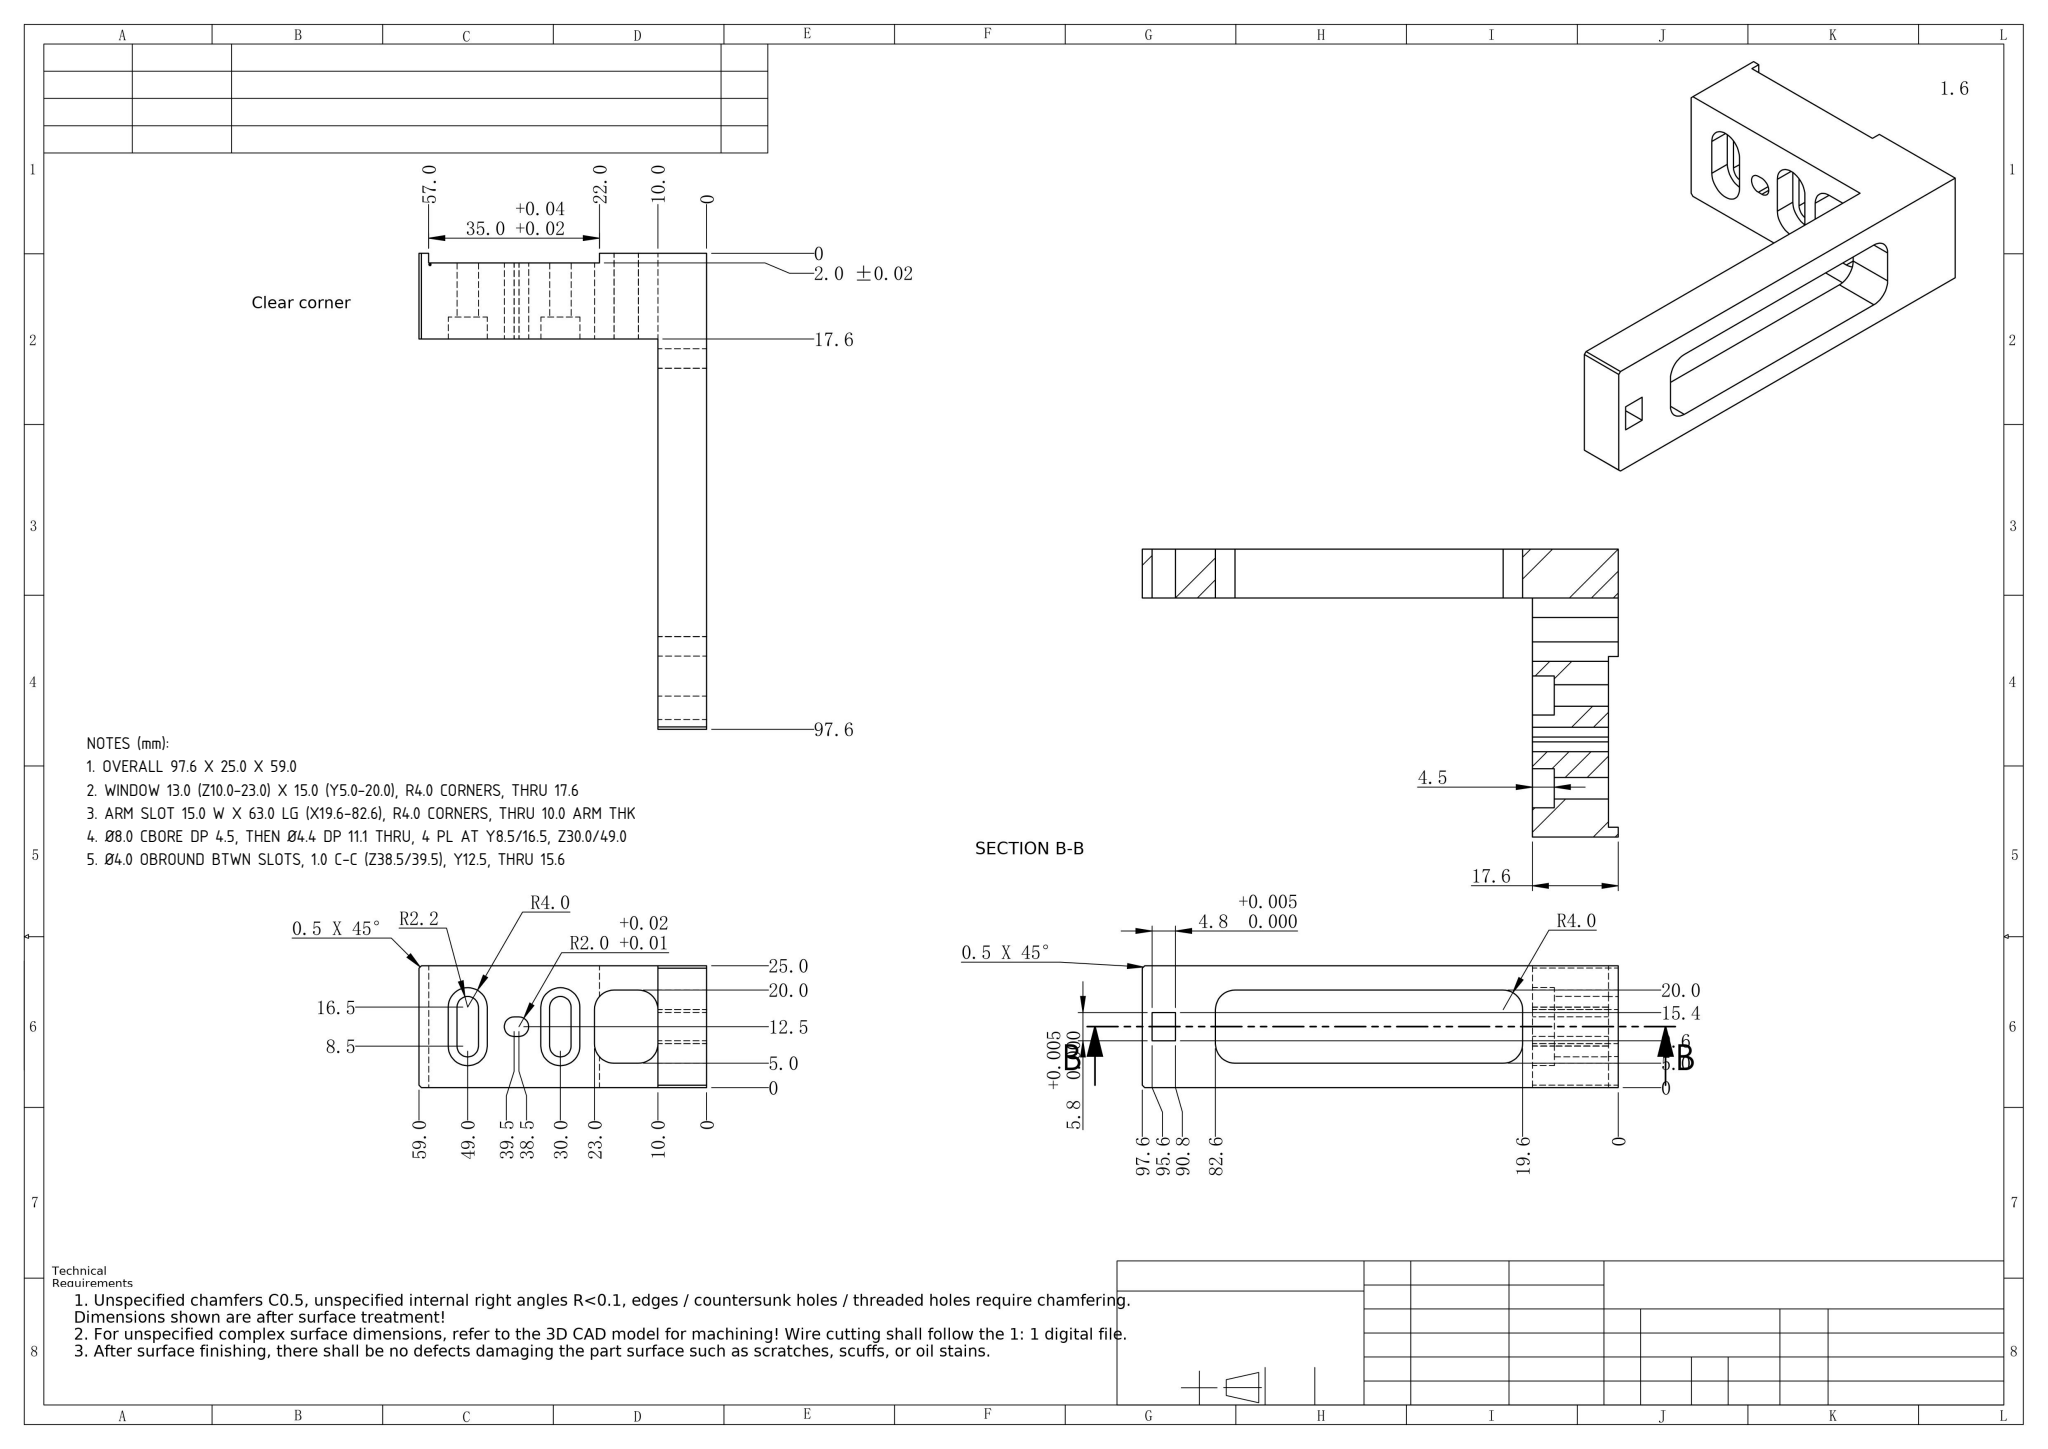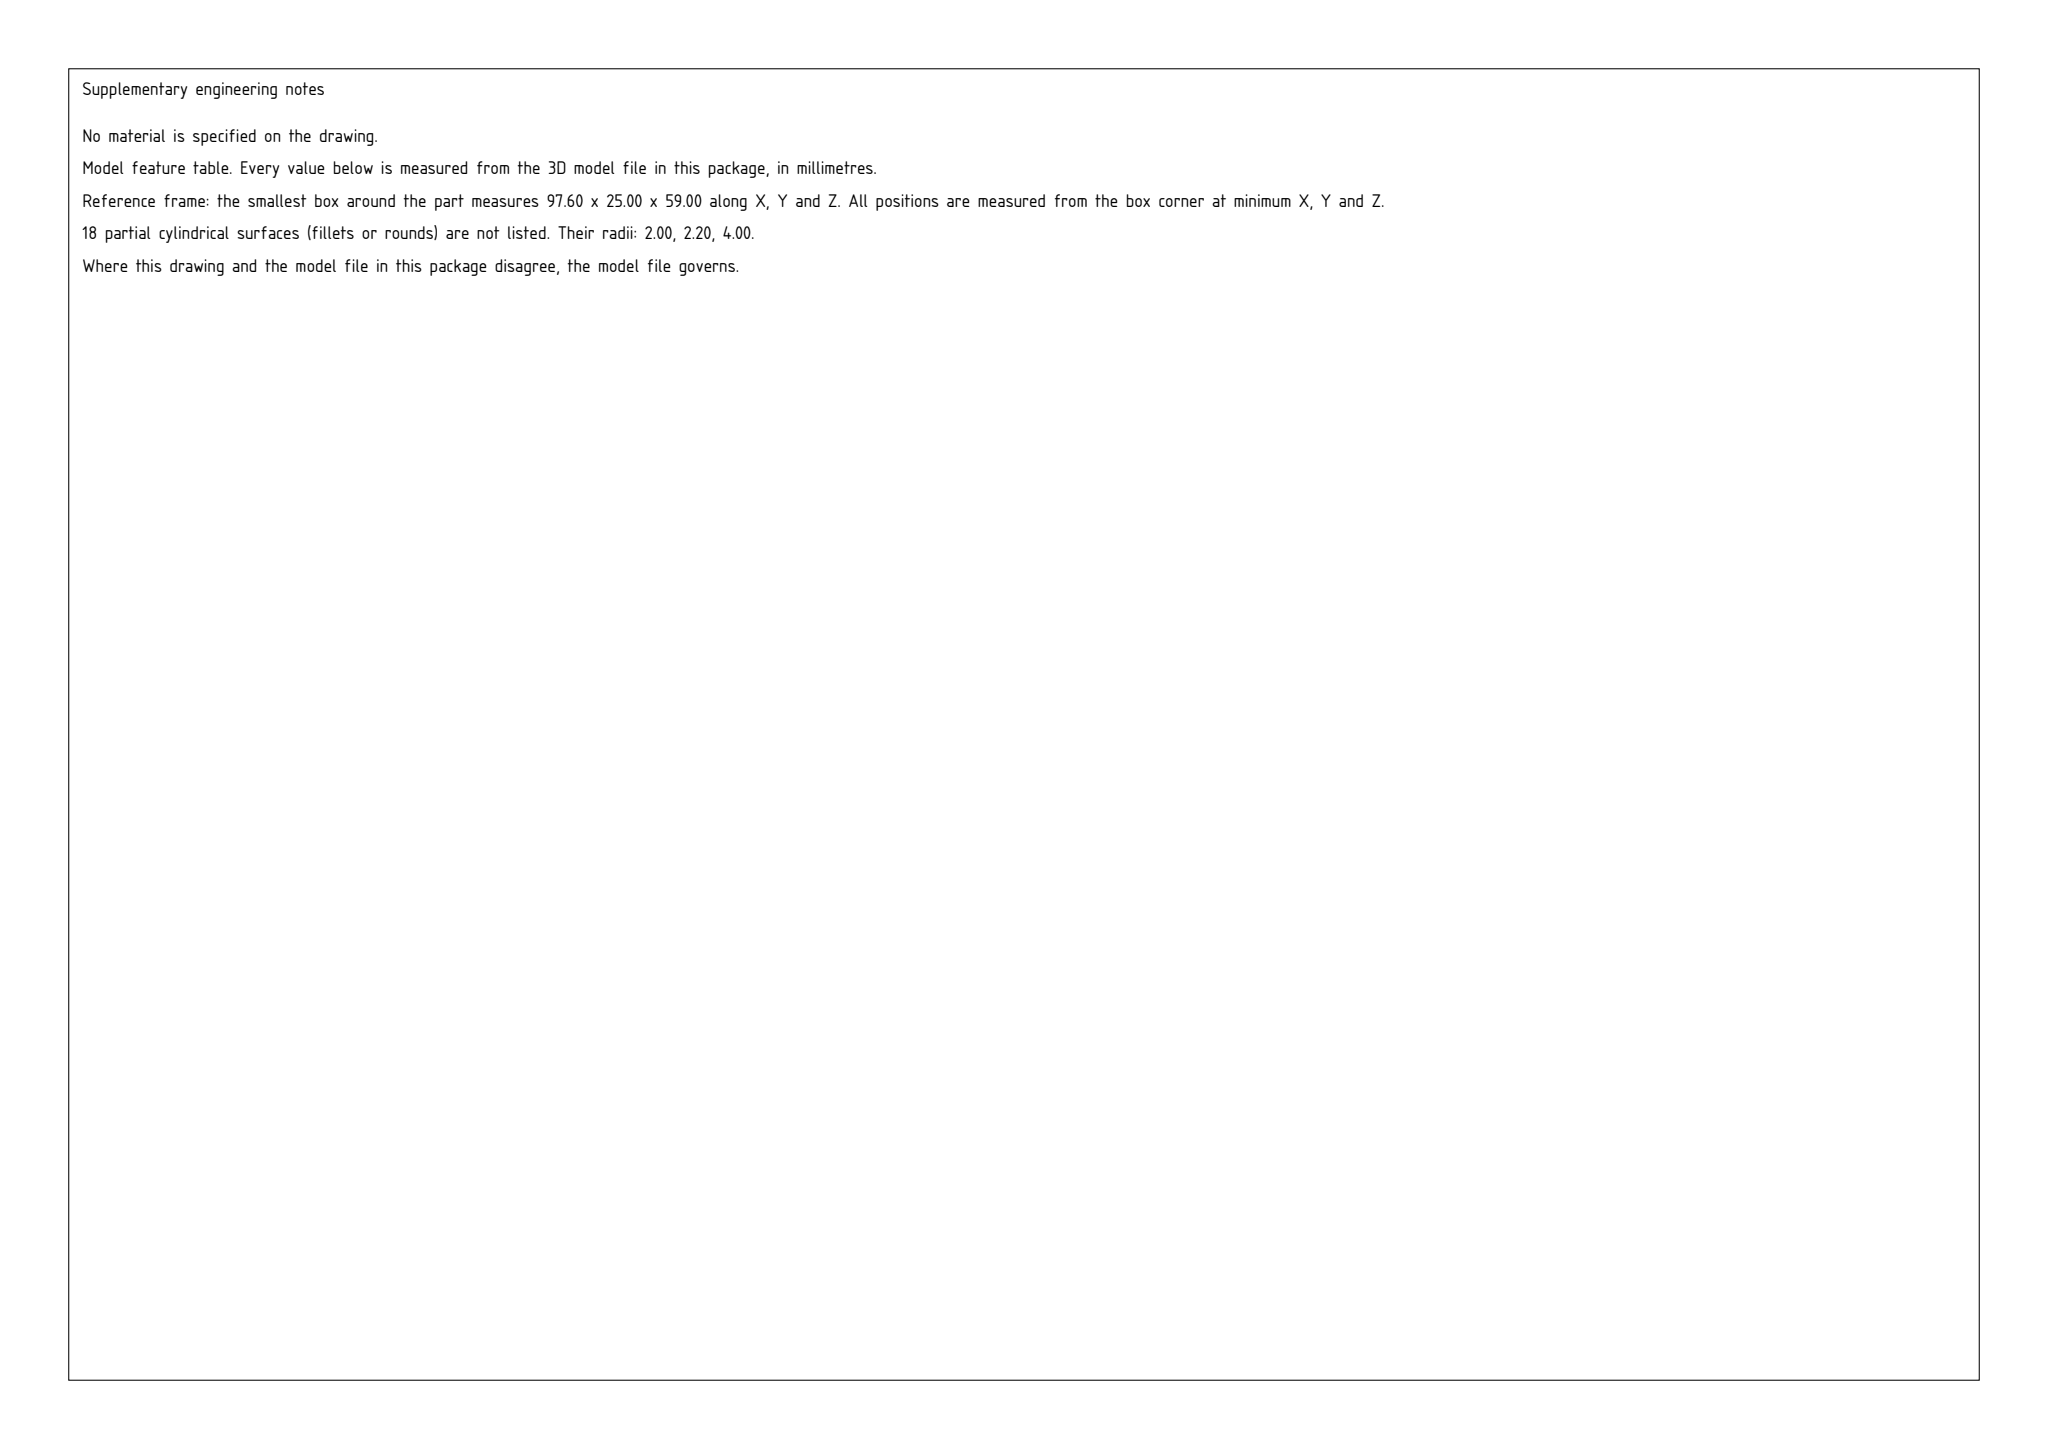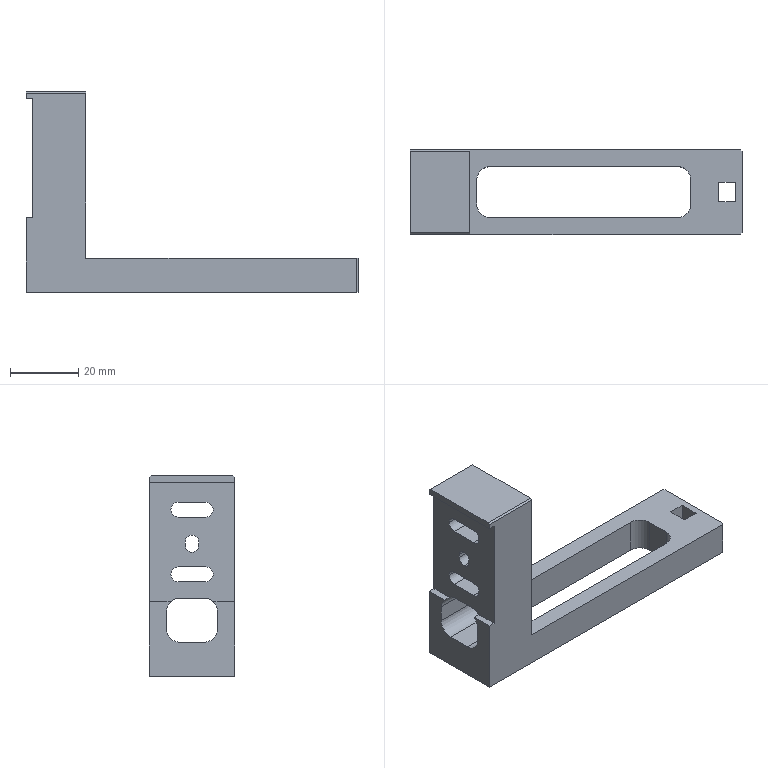Part | SolidWorks | mm | 1 solid | 63 faces | box 97.6 x 25 x 59 mm | volume 29037 mm3 | plane 40 | cylinder 23 | commonest cylinder face diameters 8 x14 4.4 x6 4 x3
Drawing notes:
OVERALL 97.6 X 25.0 X 59.0 | from the solid: bbox_xyz 97.6 x 25.0 x 59.0
WINDOW 13.0 (Z10.0-23.0) X 15.0 (Y5.0-20.0), R4.0 CORNERS, THRU 17.6 | from the solid: axis_planes z=10.0/23.0, y=5.0/20.0, x=0.0 to 17.6 thru; R4.0 corners in model
ARM SLOT 15.0 W X 63.0 LG (X19.6-82.6), R4.0 CORNERS, THRU 10.0 ARM THK | from the solid: Ø8.0 z-cyls len 10.0 at (23.6,9.0)(23.6,16.0)(78.6,9.0)(78.6,16.0); y5.0-20.0, z0-10.0
Ø8.0 CBORE DP 4.5, THEN Ø4.4 DP 11.1 THRU, 4 PL AT Y8.5/16.5, Z30.0/49.0 | from the solid: Ø8.0 x-cyl len 4.5 + Ø4.4 x-cyl len 11.1 at y8.5/16.5, z30.0/49.0; 4.5+11.1=15.6 to x17.6
Ø4.0 OBROUND BTWN SLOTS, 1.0 C-C (Z38.5/39.5), Y12.5, THRU 15.6 | from the solid: cyl Ø4.0 axis x at y12.5, z38.5 & z39.5, len 15.6 (x2.0 to x17.6)
build123d program:
from build123d import *

# Parameters (mm, degrees)
SKETCH1_W           = 97.6
SKETCH1_H           = 25
BOSS_EXTRUDE1_DEPTH = 59
SKETCH2_W           = 80
SKETCH2_H           = 25
CUT_EXTRUDE1_DEPTH  = 49
CUT_EXTRUDE3_DEPTH  = 103.499
CUT_EXTRUDE4_DEPTH  = 4.5
SKETCH6_W           = 4.8
SKETCH6_H           = 5.8
CUT_EXTRUDE5_DEPTH  = 113.035
CHAMFER1_SIZE       = 0.5
SKETCH7_W           = 2
SKETCH7_H           = 35
CUT_EXTRUDE6_DEPTH  = 117.755
SKETCH8_W           = 63
SKETCH8_H           = 15
CUT_EXTRUDE7_DEPTH  = 113.035
FILLET1_R           = 4
SKETCH9_W           = 13
SKETCH9_H           = 15
CUT_EXTRUDE8_DEPTH  = 103.499
FILLET2_R           = 4
CUT_EXTRUDE9_DEPTH  = 103.499


with BuildPart() as part:
    # Sketch1 → Boss-Extrude1 (new body)
    with BuildSketch(Plane.XY):
        with Locations((48.8, 12.5)):
            Rectangle(SKETCH1_W, SKETCH1_H)
    extrude(amount=BOSS_EXTRUDE1_DEPTH)

    # Sketch2 → Cut-Extrude1 (cut)
    with BuildSketch(Plane.XY.offset(59)):
        with Locations((57.6, 12.5)):
            Rectangle(SKETCH2_W, SKETCH2_H)
    extrude(amount=-CUT_EXTRUDE1_DEPTH, mode=Mode.SUBTRACT)

    # Sketch4 → Cut-Extrude3 (cut, through all)
    with BuildSketch(Plane(origin=(17.6, 0, 0), x_dir=(0, 0, -1), z_dir=(1, 0, 0))):
        with BuildLine():
            Line((-51.2, 8.5), (-51.2, 16.5))
            ThreePointArc((-51.2, 16.5), (-49, 18.7), (-46.8, 16.5))
            Line((-46.8, 16.5), (-46.8, 8.5))
            ThreePointArc((-46.8, 8.5), (-49, 6.3), (-51.2, 8.5))
        make_face()
        with BuildLine():
            Line((-32.2, 8.5), (-32.2, 16.5))
            ThreePointArc((-32.2, 16.5), (-30, 18.7), (-27.8, 16.5))
            Line((-27.8, 16.5), (-27.8, 8.5))
            ThreePointArc((-27.8, 8.5), (-30, 6.3), (-32.2, 8.5))
        make_face()
    extrude(amount=-CUT_EXTRUDE3_DEPTH, mode=Mode.SUBTRACT)

    # Sketch5 → Cut-Extrude4 (cut)
    with BuildSketch(Plane(origin=(17.6, 0, 0), x_dir=(0, 0, -1), z_dir=(1, 0, 0))):
        with BuildLine():
            Line((-53, 16.5), (-53, 8.5))
            ThreePointArc((-53, 8.5), (-49, 4.5), (-45, 8.5))
            Line((-45, 8.5), (-45, 16.5))
            ThreePointArc((-45, 16.5), (-49, 20.5), (-53, 16.5))
        make_face()
        with BuildLine():
            Line((-26, 8.5), (-26, 16.5))
            ThreePointArc((-26, 16.5), (-30, 20.5), (-34, 16.5))
            Line((-34, 16.5), (-34, 8.5))
            ThreePointArc((-34, 8.5), (-30, 4.5), (-26, 8.5))
        make_face()
    extrude(amount=-CUT_EXTRUDE4_DEPTH, mode=Mode.SUBTRACT)

    # Sketch6 → Cut-Extrude5 (cut, through all)
    with BuildSketch(Plane.XY.offset(10)):
        with Locations((93.2, 12.5)):
            Rectangle(SKETCH6_W, SKETCH6_H)
    extrude(amount=-CUT_EXTRUDE5_DEPTH, mode=Mode.SUBTRACT)

    # Chamfer1
    chamfer1_edges = [part.edges().sort_by_distance(p)[0] for p in [
        (8.8, 25, 59),
        (97.6, 25, 5),
        (97.6, 0, 5),
        (8.8, 0, 59),
    ]]
    chamfer(chamfer1_edges, length=CHAMFER1_SIZE)

    # Sketch7 → Cut-Extrude6 (cut, through all)
    with BuildSketch(Plane.XZ):
        with Locations((1, 39.5)):
            Rectangle(SKETCH7_W, SKETCH7_H)
    extrude(amount=-CUT_EXTRUDE6_DEPTH, mode=Mode.SUBTRACT)

    # Sketch8 → Cut-Extrude7 (cut, through all)
    with BuildSketch(Plane.XY.offset(10)):
        with Locations((51.1, 12.5)):
            Rectangle(SKETCH8_W, SKETCH8_H)
    extrude(amount=-CUT_EXTRUDE7_DEPTH, mode=Mode.SUBTRACT)

    # Fillet1
    fillet1_edges = [part.edges().sort_by_distance(p)[0] for p in [
        (19.6, 5, 5),
        (19.6, 20, 5),
        (82.6, 20, 5),
        (82.6, 5, 5),
    ]]
    fillet(fillet1_edges, radius=FILLET1_R)

    # Sketch9 → Cut-Extrude8 (cut, through all)
    with BuildSketch(Plane(origin=(17.6, 0, 0), x_dir=(0, 0, -1), z_dir=(1, 0, 0))):
        with Locations((-16.5, 12.5)):
            Rectangle(SKETCH9_W, SKETCH9_H)
    extrude(amount=-CUT_EXTRUDE8_DEPTH, mode=Mode.SUBTRACT)

    # Fillet2
    fillet2_edges = [part.edges().sort_by_distance(p)[0] for p in [
        (9.8, 5, 23),
        (9.8, 20, 23),
        (8.8, 5, 10),
        (8.8, 20, 10),
    ]]
    fillet(fillet2_edges, radius=FILLET2_R)

    # Sketch10 → Cut-Extrude9 (cut, through all)
    with BuildSketch(Plane(origin=(17.6, 0, 0), x_dir=(0, 0, -1), z_dir=(1, 0, 0))):
        with BuildLine():
            Line((-39.5, 14.5), (-38.5, 14.5))
            ThreePointArc((-38.5, 14.5), (-36.5, 12.5), (-38.5, 10.5))
            Line((-38.5, 10.5), (-39.5, 10.5))
            ThreePointArc((-39.5, 10.5), (-41.5, 12.5), (-39.5, 14.5))
        make_face()
    extrude(amount=-CUT_EXTRUDE9_DEPTH, mode=Mode.SUBTRACT)


solid = part.part